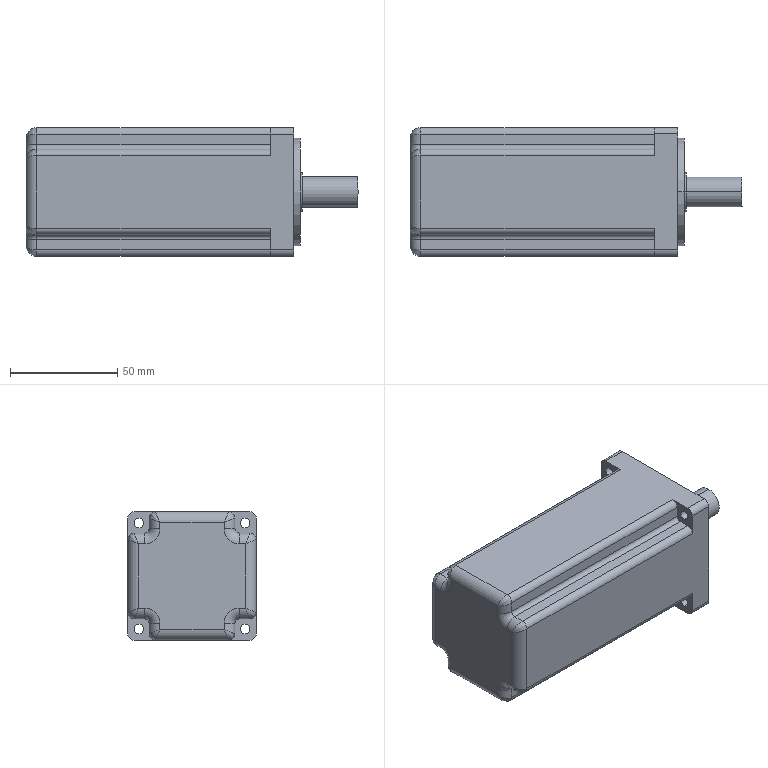Component | SolidWorks | v1ZHXTHG-KR23BSB1-1 | 1 solid | 75 faces | box 154.8 x 60 x 60 mm | volume 410503 mm3 | cylinder 42 | plane 21 | spline 8 | torus 4 | commonest cylinder face diameters 6 x12 10 x12 4.5 x8 4 x4 14 x2 18 x2 50 x2